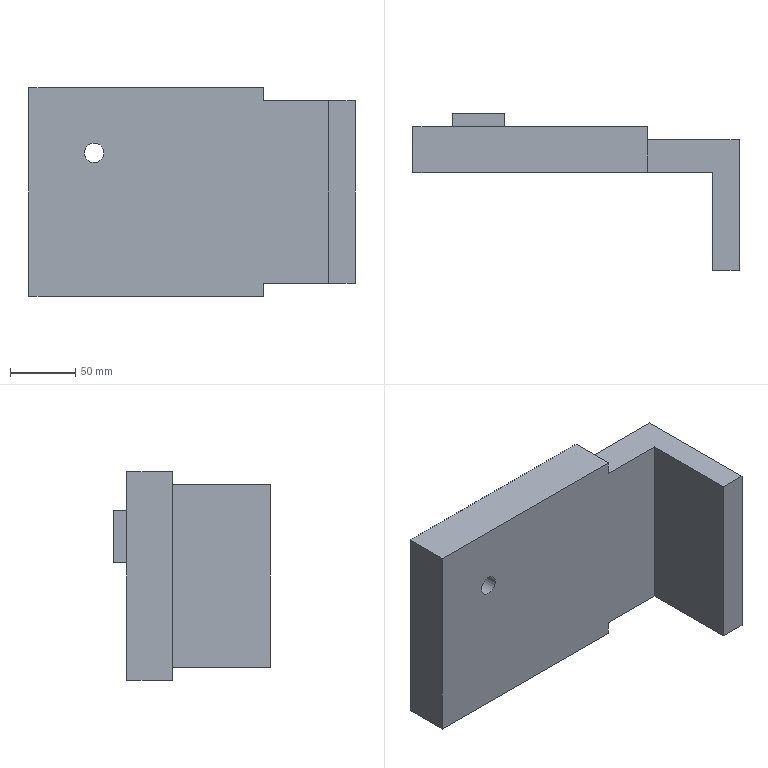Component | SolidWorks | MotorSupportPlate-1 | 1 solid | 19 faces | box 250 x 120 x 160 mm | volume 1471048 mm3 | plane 17 | cylinder 2 | commonest cylinder face diameters 15 x2
build123d program:
from build123d import *

# Parameters (mm, degrees)
SKETCH1_W                       = 20
SKETCH1_H                       = 140
BOSS_EXTRUDE1_DEPTH             = 100
SKETCH2_W                       = 25
SKETCH2_H                       = 140
BOSS_EXTRUDE2_DEPTH             = 230
BOSS_EXTRUDE3_REACH             = 482.755
SKETCH3_W                       = 180
SKETCH3_H                       = 160
BOSS_EXTRUDE3_DIRECTION_2_DEPTH = 10
SKETCH4_W                       = 40
SKETCH4_H                       = 40
SKETCH4_R                       = 7.5
BOSS_EXTRUDE4_DEPTH             = 10
CUT_EXTRUDE1_DEPTH              = 485.484
CUT_EXTRUDE1_DEPTH_BACK         = 485.484
SKETCH5_R                       = 7.5


with BuildPart() as part:
    # Sketch1 → Boss-Extrude1 (new body)
    with BuildSketch(Plane.XY):
        with Locations((455, 0)):
            Rectangle(SKETCH1_W, SKETCH1_H)
    extrude(amount=BOSS_EXTRUDE1_DEPTH)

    # Sketch2 → Boss-Extrude2 (add)
    with BuildSketch(Plane.ZY.offset(-445)):
        with Locations((87.5, 0)):
            Rectangle(SKETCH2_W, SKETCH2_H)
    extrude(amount=BOSS_EXTRUDE2_DEPTH)

    # Boss-Extrude3: up to this face of the body (flat: up to its plane)
    boss_extrude3_end = Plane(part.part.faces().sort_by_distance((330, 0, 75))[0])
    # Sketch3 → Boss-Extrude3 (add, up to the picked face)
    with BuildSketch(Plane.XY.offset(100), mode=Mode.PRIVATE) as boss_extrude3_sk1:
        with Locations((305, 0)):
            Rectangle(SKETCH3_W, SKETCH3_H)
    boss_extrude3_tool1 = split(extrude(boss_extrude3_sk1.sketch, amount=-BOSS_EXTRUDE3_REACH, mode=Mode.PRIVATE), bisect_by=boss_extrude3_end, keep=Keep.BOTH, mode=Mode.PRIVATE)
    add(boss_extrude3_tool1.solids().sort_by(Axis((305, 0, 100), (0, 0, -1)))[0])

    # Sketch3 → Boss-Extrude3 direction 2 (add)
    with BuildSketch(Plane.XY.offset(100)):
        with Locations((305, 0)):
            Rectangle(SKETCH3_W, SKETCH3_H)
    extrude(amount=BOSS_EXTRUDE3_DIRECTION_2_DEPTH)

    # Sketch4 → Boss-Extrude4 (add)
    with BuildSketch(Plane.XY.offset(110)):
        with Locations((265, -30)):
            Rectangle(SKETCH4_W, SKETCH4_H)
        with Locations((265, -30)):
            Circle(SKETCH4_R, mode=Mode.SUBTRACT)
    extrude(amount=BOSS_EXTRUDE4_DEPTH)

    # Sketch5 → Cut-Extrude1 (cut, two sides: drawn at the far end of the back side and taken through both)
    with BuildSketch(Plane.XY.offset(110).offset(-CUT_EXTRUDE1_DEPTH_BACK)):
        with Locations(Location((265, -30, 0), (0, 0, 270))):
            Circle(SKETCH5_R)
    extrude(amount=CUT_EXTRUDE1_DEPTH + CUT_EXTRUDE1_DEPTH_BACK, mode=Mode.SUBTRACT)


solid = part.part

# Placed as in the assembly
solid = solid.moved(Location((0, 150, 0), (-90, 0, 0)))
STEP:
#1=CARTESIAN_POINT('',(10.138,10.63,1.181));
#2=VERTEX_POINT('',#1);
#3=CARTESIAN_POINT('',(10.728,10.63,1.181));
#4=VERTEX_POINT('',#3);
#5=CARTESIAN_POINT('',(10.433,10.63,1.181));
#6=DIRECTION('',(0.,1.,0.));
#7=DIRECTION('',(1.,0.,0.));
#8=AXIS2_PLACEMENT_3D('',#5,#6,#7);
#9=CIRCLE('',#8,0.2953);
#10=EDGE_CURVE('',#2,#4,#9,.T.);
#11=ORIENTED_EDGE('',*,*,#10,.T.);
#12=CARTESIAN_POINT('',(10.728,8.858,1.181));
#13=VERTEX_POINT('',#12);
#14=CARTESIAN_POINT('',(10.728,10.63,1.181));
#15=DIRECTION('',(0.,-1.,0.));
#16=VECTOR('',#15,39.37);
#17=LINE('',#14,#16);
#18=EDGE_CURVE('',#4,#13,#17,.T.);
#19=ORIENTED_EDGE('',*,*,#18,.T.);
#20=CARTESIAN_POINT('',(10.138,8.858,1.181));
#21=VERTEX_POINT('',#20);
#22=CARTESIAN_POINT('',(10.433,8.858,1.181));
#23=DIRECTION('',(0.,1.,-0.));
#24=DIRECTION('',(0.,0.,1.));
#25=AXIS2_PLACEMENT_3D('',#22,#23,#24);
#26=CIRCLE('',#25,0.2953);
#27=EDGE_CURVE('',#21,#13,#26,.T.);
#28=ORIENTED_EDGE('',*,*,#27,.F.);
#29=CARTESIAN_POINT('',(10.138,10.63,1.181));
#30=DIRECTION('',(0.,-1.,0.));
#31=VECTOR('',#30,39.37);
#32=LINE('',#29,#31);
#33=EDGE_CURVE('',#2,#21,#32,.T.);
#34=ORIENTED_EDGE('',*,*,#33,.F.);
#35=EDGE_LOOP('',(#11,#19,#28,#34));
#36=FACE_OUTER_BOUND('',#35,.T.);
#37=CARTESIAN_POINT('',(10.433,10.63,1.181));
#38=DIRECTION('',(0.,-1.,0.));
#39=DIRECTION('',(-1.,0.,0.));
#40=AXIS2_PLACEMENT_3D('',#37,#38,#39);
#41=CYLINDRICAL_SURFACE('',#40,0.2953);
#42=ADVANCED_FACE('',(#36),#41,.F.);
#43=CARTESIAN_POINT('',(15.551,9.843,-2.756));
#44=VERTEX_POINT('',#43);
#45=CARTESIAN_POINT('',(15.551,8.858,-2.756));
#46=VERTEX_POINT('',#45);
#47=CARTESIAN_POINT('',(15.551,9.843,-2.756));
#48=DIRECTION('',(0.,-1.,0.));
#49=VECTOR('',#48,39.37);
#50=LINE('',#47,#49);
#51=EDGE_CURVE('',#44,#46,#50,.T.);
#52=ORIENTED_EDGE('',*,*,#51,.F.);
#53=CARTESIAN_POINT('',(18.307,9.843,-2.756));
#54=VERTEX_POINT('',#53);
#55=CARTESIAN_POINT('',(18.307,9.843,-2.756));
#56=DIRECTION('',(-1.,0.,0.));
#57=VECTOR('',#56,39.37);
#58=LINE('',#55,#57);
#59=EDGE_CURVE('',#54,#44,#58,.T.);
#60=ORIENTED_EDGE('',*,*,#59,.F.);
#61=CARTESIAN_POINT('',(18.307,5.906,-2.756));
#62=VERTEX_POINT('',#61);
#63=CARTESIAN_POINT('',(18.307,9.843,-2.756));
#64=DIRECTION('',(0.,-1.,0.));
#65=VECTOR('',#64,39.37);
#66=LINE('',#63,#65);
#67=EDGE_CURVE('',#54,#62,#66,.T.);
#68=ORIENTED_EDGE('',*,*,#67,.T.);
#69=CARTESIAN_POINT('',(17.52,5.906,-2.756));
#70=VERTEX_POINT('',#69);
#71=CARTESIAN_POINT('',(18.307,5.906,-2.756));
#72=DIRECTION('',(-1.,0.,0.));
#73=VECTOR('',#72,39.37);
#74=LINE('',#71,#73);
#75=EDGE_CURVE('',#62,#70,#74,.T.);
#76=ORIENTED_EDGE('',*,*,#75,.T.);
#77=CARTESIAN_POINT('',(17.52,8.858,-2.756));
#78=VERTEX_POINT('',#77);
#79=CARTESIAN_POINT('',(17.52,9.843,-2.756));
#80=DIRECTION('',(0.,-1.,0.));
#81=VECTOR('',#80,39.37);
#82=LINE('',#79,#81);
#83=EDGE_CURVE('',#78,#70,#82,.T.);
#84=ORIENTED_EDGE('',*,*,#83,.F.);
#85=CARTESIAN_POINT('',(8.465,8.858,-2.756));
#86=DIRECTION('',(1.,0.,0.));
#87=VECTOR('',#86,39.37);
#88=LINE('',#85,#87);
#89=EDGE_CURVE('',#46,#78,#88,.T.);
#90=ORIENTED_EDGE('',*,*,#89,.F.);
#91=EDGE_LOOP('',(#52,#60,#68,#76,#84,#90));
#92=FACE_OUTER_BOUND('',#91,.T.);
#93=CARTESIAN_POINT('',(18.307,9.843,-2.756));
#94=DIRECTION('',(0.,0.,1.));
#95=DIRECTION('',(0.,-1.,0.));
#96=AXIS2_PLACEMENT_3D('',#93,#94,#95);
#97=PLANE('',#96);
#98=ADVANCED_FACE('',(#92),#97,.F.);
#99=CARTESIAN_POINT('',(15.551,8.858,2.756));
#100=VERTEX_POINT('',#99);
#101=CARTESIAN_POINT('',(15.551,9.843,2.756));
#102=VERTEX_POINT('',#101);
#103=CARTESIAN_POINT('',(15.551,9.843,2.756));
#104=DIRECTION('',(0.,1.,0.));
#105=VECTOR('',#104,39.37);
#106=LINE('',#103,#105);
#107=EDGE_CURVE('',#100,#102,#106,.T.);
#108=ORIENTED_EDGE('',*,*,#107,.F.);
#109=CARTESIAN_POINT('',(17.52,8.858,2.756));
#110=VERTEX_POINT('',#109);
#111=CARTESIAN_POINT('',(8.465,8.858,2.756));
#112=DIRECTION('',(1.,0.,0.));
#113=VECTOR('',#112,39.37);
#114=LINE('',#111,#113);
#115=EDGE_CURVE('',#100,#110,#114,.T.);
#116=ORIENTED_EDGE('',*,*,#115,.T.);
#117=CARTESIAN_POINT('',(17.52,5.906,2.756));
#118=VERTEX_POINT('',#117);
#119=CARTESIAN_POINT('',(17.52,9.843,2.756));
#120=DIRECTION('',(0.,-1.,0.));
#121=VECTOR('',#120,39.37);
#122=LINE('',#119,#121);
#123=EDGE_CURVE('',#110,#118,#122,.T.);
#124=ORIENTED_EDGE('',*,*,#123,.T.);
#125=CARTESIAN_POINT('',(18.307,5.906,2.756));
#126=VERTEX_POINT('',#125);
#127=CARTESIAN_POINT('',(18.307,5.906,2.756));
#128=DIRECTION('',(1.,0.,0.));
#129=VECTOR('',#128,39.37);
#130=LINE('',#127,#129);
#131=EDGE_CURVE('',#118,#126,#130,.T.);
#132=ORIENTED_EDGE('',*,*,#131,.T.);
#133=CARTESIAN_POINT('',(18.307,9.843,2.756));
#134=VERTEX_POINT('',#133);
#135=CARTESIAN_POINT('',(18.307,9.843,2.756));
#136=DIRECTION('',(0.,-1.,0.));
#137=VECTOR('',#136,39.37);
#138=LINE('',#135,#137);
#139=EDGE_CURVE('',#134,#126,#138,.T.);
#140=ORIENTED_EDGE('',*,*,#139,.F.);
#141=CARTESIAN_POINT('',(18.307,9.843,2.756));
#142=DIRECTION('',(1.,0.,0.));
#143=VECTOR('',#142,39.37);
#144=LINE('',#141,#143);
#145=EDGE_CURVE('',#102,#134,#144,.T.);
#146=ORIENTED_EDGE('',*,*,#145,.F.);
#147=EDGE_LOOP('',(#108,#116,#124,#132,#140,#146));
#148=FACE_OUTER_BOUND('',#147,.T.);
#149=CARTESIAN_POINT('',(18.307,9.843,2.756));
#150=DIRECTION('',(0.,0.,-1.));
#151=DIRECTION('',(-1.,0.,-0.));
#152=AXIS2_PLACEMENT_3D('',#149,#150,#151);
#153=PLANE('',#152);
#154=ADVANCED_FACE('',(#148),#153,.F.);
#155=ORIENTED_EDGE('',*,*,#59,.T.);
#156=CARTESIAN_POINT('',(15.551,9.843,0.));
#157=DIRECTION('',(0.,0.,1.));
#158=VECTOR('',#157,39.37);
#159=LINE('',#156,#158);
#160=EDGE_CURVE('',#44,#102,#159,.T.);
#161=ORIENTED_EDGE('',*,*,#160,.T.);
#162=ORIENTED_EDGE('',*,*,#145,.T.);
#163=CARTESIAN_POINT('',(18.307,9.843,2.756));
#164=DIRECTION('',(0.,0.,-1.));
#165=VECTOR('',#164,39.37);
#166=LINE('',#163,#165);
#167=EDGE_CURVE('',#134,#54,#166,.T.);
#168=ORIENTED_EDGE('',*,*,#167,.T.);
#169=EDGE_LOOP('',(#155,#161,#162,#168));
#170=FACE_OUTER_BOUND('',#169,.T.);
#171=CARTESIAN_POINT('',(0.,9.843,0.));
#172=DIRECTION('',(0.,1.,0.));
#173=DIRECTION('',(1.,0.,0.));
#174=AXIS2_PLACEMENT_3D('',#171,#172,#173);
#175=PLANE('',#174);
#176=ADVANCED_FACE('',(#170),#175,.T.);
#177=CARTESIAN_POINT('',(17.52,8.858,-2.756));
#178=DIRECTION('',(0.,0.,1.));
#179=VECTOR('',#178,39.37);
#180=LINE('',#177,#179);
#181=EDGE_CURVE('',#78,#110,#180,.T.);
#182=ORIENTED_EDGE('',*,*,#181,.F.);
#183=ORIENTED_EDGE('',*,*,#83,.T.);
#184=CARTESIAN_POINT('',(17.52,5.906,2.756));
#185=DIRECTION('',(0.,0.,1.));
#186=VECTOR('',#185,39.37);
#187=LINE('',#184,#186);
#188=EDGE_CURVE('',#70,#118,#187,.T.);
#189=ORIENTED_EDGE('',*,*,#188,.T.);
#190=ORIENTED_EDGE('',*,*,#123,.F.);
#191=EDGE_LOOP('',(#182,#183,#189,#190));
#192=FACE_OUTER_BOUND('',#191,.T.);
#193=CARTESIAN_POINT('',(17.52,9.843,2.756));
#194=DIRECTION('',(1.,0.,0.));
#195=DIRECTION('',(0.,-1.,0.));
#196=AXIS2_PLACEMENT_3D('',#193,#194,#195);
#197=PLANE('',#196);
#198=ADVANCED_FACE('',(#192),#197,.F.);
#199=CARTESIAN_POINT('',(18.307,5.906,2.756));
#200=DIRECTION('',(0.,0.,-1.));
#201=VECTOR('',#200,39.37);
#202=LINE('',#199,#201);
#203=EDGE_CURVE('',#126,#62,#202,.T.);
#204=ORIENTED_EDGE('',*,*,#203,.T.);
#205=ORIENTED_EDGE('',*,*,#67,.F.);
#206=ORIENTED_EDGE('',*,*,#167,.F.);
#207=ORIENTED_EDGE('',*,*,#139,.T.);
#208=EDGE_LOOP('',(#204,#205,#206,#207));
#209=FACE_OUTER_BOUND('',#208,.T.);
#210=CARTESIAN_POINT('',(18.307,9.843,2.756));
#211=DIRECTION('',(-1.,0.,0.));
#212=DIRECTION('',(0.,1.,0.));
#213=AXIS2_PLACEMENT_3D('',#210,#211,#212);
#214=PLANE('',#213);
#215=ADVANCED_FACE('',(#209),#214,.F.);
#216=ORIENTED_EDGE('',*,*,#203,.F.);
#217=ORIENTED_EDGE('',*,*,#131,.F.);
#218=ORIENTED_EDGE('',*,*,#188,.F.);
#219=ORIENTED_EDGE('',*,*,#75,.F.);
#220=EDGE_LOOP('',(#216,#217,#218,#219));
#221=FACE_OUTER_BOUND('',#220,.T.);
#222=CARTESIAN_POINT('',(0.,5.906,0.));
#223=DIRECTION('',(0.,1.,0.));
#224=DIRECTION('',(1.,0.,0.));
#225=AXIS2_PLACEMENT_3D('',#222,#223,#224);
#226=PLANE('',#225);
#227=ADVANCED_FACE('',(#221),#226,.F.);
#228=ORIENTED_EDGE('',*,*,#27,.T.);
#229=CARTESIAN_POINT('',(10.433,8.858,1.181));
#230=DIRECTION('',(0.,1.,-0.));
#231=DIRECTION('',(0.,0.,1.));
#232=AXIS2_PLACEMENT_3D('',#229,#230,#231);
#233=CIRCLE('',#232,0.2953);
#234=EDGE_CURVE('',#13,#21,#233,.T.);
#235=ORIENTED_EDGE('',*,*,#234,.T.);
#236=EDGE_LOOP('',(#228,#235));
#237=FACE_BOUND('',#236,.T.);
#238=CARTESIAN_POINT('',(8.465,8.858,-3.15));
#239=VERTEX_POINT('',#238);
#240=CARTESIAN_POINT('',(8.465,8.858,3.15));
#241=VERTEX_POINT('',#240);
#242=CARTESIAN_POINT('',(8.465,8.858,-2.756));
#243=DIRECTION('',(0.,0.,1.));
#244=VECTOR('',#243,39.37);
#245=LINE('',#242,#244);
#246=EDGE_CURVE('',#239,#241,#245,.T.);
#247=ORIENTED_EDGE('',*,*,#246,.F.);
#248=CARTESIAN_POINT('',(15.551,8.858,-3.15));
#249=VERTEX_POINT('',#248);
#250=CARTESIAN_POINT('',(8.465,8.858,-3.15));
#251=DIRECTION('',(1.,0.,0.));
#252=VECTOR('',#251,39.37);
#253=LINE('',#250,#252);
#254=EDGE_CURVE('',#239,#249,#253,.T.);
#255=ORIENTED_EDGE('',*,*,#254,.T.);
#256=CARTESIAN_POINT('',(15.551,8.858,-3.15));
#257=DIRECTION('',(0.,0.,1.));
#258=VECTOR('',#257,39.37);
#259=LINE('',#256,#258);
#260=EDGE_CURVE('',#249,#46,#259,.T.);
#261=ORIENTED_EDGE('',*,*,#260,.T.);
#262=ORIENTED_EDGE('',*,*,#89,.T.);
#263=ORIENTED_EDGE('',*,*,#181,.T.);
#264=ORIENTED_EDGE('',*,*,#115,.F.);
#265=CARTESIAN_POINT('',(15.551,8.858,3.15));
#266=VERTEX_POINT('',#265);
#267=CARTESIAN_POINT('',(15.551,8.858,-3.15));
#268=DIRECTION('',(0.,0.,1.));
#269=VECTOR('',#268,39.37);
#270=LINE('',#267,#269);
#271=EDGE_CURVE('',#100,#266,#270,.T.);
#272=ORIENTED_EDGE('',*,*,#271,.T.);
#273=CARTESIAN_POINT('',(8.465,8.858,3.15));
#274=DIRECTION('',(-1.,0.,0.));
#275=VECTOR('',#274,39.37);
#276=LINE('',#273,#275);
#277=EDGE_CURVE('',#266,#241,#276,.T.);
#278=ORIENTED_EDGE('',*,*,#277,.T.);
#279=EDGE_LOOP('',(#247,#255,#261,#262,#263,#264,#272,#278));
#280=FACE_OUTER_BOUND('',#279,.T.);
#281=CARTESIAN_POINT('',(8.465,8.858,-2.756));
#282=DIRECTION('',(0.,1.,-0.));
#283=DIRECTION('',(0.,0.,1.));
#284=AXIS2_PLACEMENT_3D('',#281,#282,#283);
#285=PLANE('',#284);
#286=ADVANCED_FACE('',(#237,#280),#285,.F.);
#287=CARTESIAN_POINT('',(8.465,10.236,-3.15));
#288=VERTEX_POINT('',#287);
#289=CARTESIAN_POINT('',(8.465,10.236,-3.15));
#290=DIRECTION('',(0.,-1.,0.));
#291=VECTOR('',#290,39.37);
#292=LINE('',#289,#291);
#293=EDGE_CURVE('',#288,#239,#292,.T.);
#294=ORIENTED_EDGE('',*,*,#293,.T.);
#295=ORIENTED_EDGE('',*,*,#246,.T.);
#296=CARTESIAN_POINT('',(8.465,10.236,3.15));
#297=VERTEX_POINT('',#296);
#298=CARTESIAN_POINT('',(8.465,10.236,3.15));
#299=DIRECTION('',(0.,-1.,0.));
#300=VECTOR('',#299,39.37);
#301=LINE('',#298,#300);
#302=EDGE_CURVE('',#297,#241,#301,.T.);
#303=ORIENTED_EDGE('',*,*,#302,.F.);
#304=CARTESIAN_POINT('',(8.465,10.236,-3.15));
#305=DIRECTION('',(0.,0.,1.));
#306=VECTOR('',#305,39.37);
#307=LINE('',#304,#306);
#308=EDGE_CURVE('',#288,#297,#307,.T.);
#309=ORIENTED_EDGE('',*,*,#308,.F.);
#310=EDGE_LOOP('',(#294,#295,#303,#309));
#311=FACE_OUTER_BOUND('',#310,.T.);
#312=CARTESIAN_POINT('',(8.465,5.906,0.));
#313=DIRECTION('',(1.,0.,0.));
#314=DIRECTION('',(0.,-1.,0.));
#315=AXIS2_PLACEMENT_3D('',#312,#313,#314);
#316=PLANE('',#315);
#317=ADVANCED_FACE('',(#311),#316,.F.);
#318=ORIENTED_EDGE('',*,*,#160,.F.);
#319=ORIENTED_EDGE('',*,*,#51,.T.);
#320=ORIENTED_EDGE('',*,*,#260,.F.);
#321=CARTESIAN_POINT('',(15.551,10.236,-3.15));
#322=VERTEX_POINT('',#321);
#323=CARTESIAN_POINT('',(15.551,10.236,-3.15));
#324=DIRECTION('',(0.,-1.,0.));
#325=VECTOR('',#324,39.37);
#326=LINE('',#323,#325);
#327=EDGE_CURVE('',#322,#249,#326,.T.);
#328=ORIENTED_EDGE('',*,*,#327,.F.);
#329=CARTESIAN_POINT('',(15.551,10.236,3.15));
#330=VERTEX_POINT('',#329);
#331=CARTESIAN_POINT('',(15.551,10.236,-3.15));
#332=DIRECTION('',(0.,0.,-1.));
#333=VECTOR('',#332,39.37);
#334=LINE('',#331,#333);
#335=EDGE_CURVE('',#330,#322,#334,.T.);
#336=ORIENTED_EDGE('',*,*,#335,.F.);
#337=CARTESIAN_POINT('',(15.551,10.236,3.15));
#338=DIRECTION('',(0.,-1.,0.));
#339=VECTOR('',#338,39.37);
#340=LINE('',#337,#339);
#341=EDGE_CURVE('',#330,#266,#340,.T.);
#342=ORIENTED_EDGE('',*,*,#341,.T.);
#343=ORIENTED_EDGE('',*,*,#271,.F.);
#344=ORIENTED_EDGE('',*,*,#107,.T.);
#345=EDGE_LOOP('',(#318,#319,#320,#328,#336,#342,#343,#344));
#346=FACE_OUTER_BOUND('',#345,.T.);
#347=CARTESIAN_POINT('',(15.551,10.236,-3.15));
#348=DIRECTION('',(-1.,0.,0.));
#349=DIRECTION('',(0.,1.,0.));
#350=AXIS2_PLACEMENT_3D('',#347,#348,#349);
#351=PLANE('',#350);
#352=ADVANCED_FACE('',(#346),#351,.F.);
#353=ORIENTED_EDGE('',*,*,#302,.T.);
#354=ORIENTED_EDGE('',*,*,#277,.F.);
#355=ORIENTED_EDGE('',*,*,#341,.F.);
#356=CARTESIAN_POINT('',(8.465,10.236,3.15));
#357=DIRECTION('',(1.,0.,-0.));
#358=VECTOR('',#357,39.37);
#359=LINE('',#356,#358);
#360=EDGE_CURVE('',#297,#330,#359,.T.);
#361=ORIENTED_EDGE('',*,*,#360,.F.);
#362=EDGE_LOOP('',(#353,#354,#355,#361));
#363=FACE_OUTER_BOUND('',#362,.T.);
#364=CARTESIAN_POINT('',(8.465,10.236,3.15));
#365=DIRECTION('',(-0.,0.,-1.));
#366=DIRECTION('',(-1.,0.,0.));
#367=AXIS2_PLACEMENT_3D('',#364,#365,#366);
#368=PLANE('',#367);
#369=ADVANCED_FACE('',(#363),#368,.F.);
#370=ORIENTED_EDGE('',*,*,#327,.T.);
#371=ORIENTED_EDGE('',*,*,#254,.F.);
#372=ORIENTED_EDGE('',*,*,#293,.F.);
#373=CARTESIAN_POINT('',(8.465,10.236,-3.15));
#374=DIRECTION('',(-1.,0.,0.));
#375=VECTOR('',#374,39.37);
#376=LINE('',#373,#375);
#377=EDGE_CURVE('',#322,#288,#376,.T.);
#378=ORIENTED_EDGE('',*,*,#377,.F.);
#379=EDGE_LOOP('',(#370,#371,#372,#378));
#380=FACE_OUTER_BOUND('',#379,.T.);
#381=CARTESIAN_POINT('',(8.465,10.236,-3.15));
#382=DIRECTION('',(0.,0.,1.));
#383=DIRECTION('',(0.,-1.,0.));
#384=AXIS2_PLACEMENT_3D('',#381,#382,#383);
#385=PLANE('',#384);
#386=ADVANCED_FACE('',(#380),#385,.F.);
#387=CARTESIAN_POINT('',(11.22,10.236,0.3937));
#388=VERTEX_POINT('',#387);
#389=CARTESIAN_POINT('',(9.646,10.236,0.3937));
#390=VERTEX_POINT('',#389);
#391=CARTESIAN_POINT('',(9.646,10.236,0.3937));
#392=DIRECTION('',(-1.,0.,0.));
#393=VECTOR('',#392,39.37);
#394=LINE('',#391,#393);
#395=EDGE_CURVE('',#388,#390,#394,.T.);
#396=ORIENTED_EDGE('',*,*,#395,.F.);
#397=CARTESIAN_POINT('',(11.22,10.236,1.969));
#398=VERTEX_POINT('',#397);
#399=CARTESIAN_POINT('',(11.22,10.236,0.3937));
#400=DIRECTION('',(0.,0.,-1.));
#401=VECTOR('',#400,39.37);
#402=LINE('',#399,#401);
#403=EDGE_CURVE('',#398,#388,#402,.T.);
#404=ORIENTED_EDGE('',*,*,#403,.F.);
#405=CARTESIAN_POINT('',(9.646,10.236,1.969));
#406=VERTEX_POINT('',#405);
#407=CARTESIAN_POINT('',(9.646,10.236,1.969));
#408=DIRECTION('',(1.,0.,0.));
#409=VECTOR('',#408,39.37);
#410=LINE('',#407,#409);
#411=EDGE_CURVE('',#406,#398,#410,.T.);
#412=ORIENTED_EDGE('',*,*,#411,.F.);
#413=CARTESIAN_POINT('',(9.646,10.236,0.3937));
#414=DIRECTION('',(0.,0.,1.));
#415=VECTOR('',#414,39.37);
#416=LINE('',#413,#415);
#417=EDGE_CURVE('',#390,#406,#416,.T.);
#418=ORIENTED_EDGE('',*,*,#417,.F.);
#419=EDGE_LOOP('',(#396,#404,#412,#418));
#420=FACE_BOUND('',#419,.T.);
#421=ORIENTED_EDGE('',*,*,#308,.T.);
#422=ORIENTED_EDGE('',*,*,#360,.T.);
#423=ORIENTED_EDGE('',*,*,#335,.T.);
#424=ORIENTED_EDGE('',*,*,#377,.T.);
#425=EDGE_LOOP('',(#421,#422,#423,#424));
#426=FACE_OUTER_BOUND('',#425,.T.);
#427=CARTESIAN_POINT('',(0.,10.236,0.));
#428=DIRECTION('',(0.,1.,0.));
#429=DIRECTION('',(1.,0.,0.));
#430=AXIS2_PLACEMENT_3D('',#427,#428,#429);
#431=PLANE('',#430);
#432=ADVANCED_FACE('',(#420,#426),#431,.T.);
#433=CARTESIAN_POINT('',(11.22,10.63,1.969));
#434=VERTEX_POINT('',#433);
#435=CARTESIAN_POINT('',(11.22,10.63,0.3937));
#436=VERTEX_POINT('',#435);
#437=CARTESIAN_POINT('',(11.22,10.63,0.3937));
#438=DIRECTION('',(0.,0.,-1.));
#439=VECTOR('',#438,39.37);
#440=LINE('',#437,#439);
#441=EDGE_CURVE('',#434,#436,#440,.T.);
#442=ORIENTED_EDGE('',*,*,#441,.T.);
#443=CARTESIAN_POINT('',(9.646,10.63,0.3937));
#444=VERTEX_POINT('',#443);
#445=CARTESIAN_POINT('',(9.646,10.63,0.3937));
#446=DIRECTION('',(-1.,0.,0.));
#447=VECTOR('',#446,39.37);
#448=LINE('',#445,#447);
#449=EDGE_CURVE('',#436,#444,#448,.T.);
#450=ORIENTED_EDGE('',*,*,#449,.T.);
#451=CARTESIAN_POINT('',(9.646,10.63,1.969));
#452=VERTEX_POINT('',#451);
#453=CARTESIAN_POINT('',(9.646,10.63,0.3937));
#454=DIRECTION('',(0.,0.,1.));
#455=VECTOR('',#454,39.37);
#456=LINE('',#453,#455);
#457=EDGE_CURVE('',#444,#452,#456,.T.);
#458=ORIENTED_EDGE('',*,*,#457,.T.);
#459=CARTESIAN_POINT('',(9.646,10.63,1.969));
#460=DIRECTION('',(1.,0.,0.));
#461=VECTOR('',#460,39.37);
#462=LINE('',#459,#461);
#463=EDGE_CURVE('',#452,#434,#462,.T.);
#464=ORIENTED_EDGE('',*,*,#463,.T.);
#465=EDGE_LOOP('',(#442,#450,#458,#464));
#466=FACE_OUTER_BOUND('',#465,.T.);
#467=ORIENTED_EDGE('',*,*,#10,.F.);
#468=CARTESIAN_POINT('',(10.433,10.63,1.181));
#469=DIRECTION('',(0.,1.,0.));
#470=DIRECTION('',(1.,0.,0.));
#471=AXIS2_PLACEMENT_3D('',#468,#469,#470);
#472=CIRCLE('',#471,0.2953);
#473=EDGE_CURVE('',#4,#2,#472,.T.);
#474=ORIENTED_EDGE('',*,*,#473,.F.);
#475=EDGE_LOOP('',(#467,#474));
#476=FACE_BOUND('',#475,.T.);
#477=CARTESIAN_POINT('',(0.,10.63,0.));
#478=DIRECTION('',(0.,1.,0.));
#479=DIRECTION('',(1.,0.,0.));
#480=AXIS2_PLACEMENT_3D('',#477,#478,#479);
#481=PLANE('',#480);
#482=ADVANCED_FACE('',(#466,#476),#481,.T.);
#483=ORIENTED_EDGE('',*,*,#403,.T.);
#484=CARTESIAN_POINT('',(11.22,10.63,0.3937));
#485=DIRECTION('',(0.,-1.,0.));
#486=VECTOR('',#485,39.37);
#487=LINE('',#484,#486);
#488=EDGE_CURVE('',#436,#388,#487,.T.);
#489=ORIENTED_EDGE('',*,*,#488,.F.);
#490=ORIENTED_EDGE('',*,*,#441,.F.);
#491=CARTESIAN_POINT('',(11.22,10.63,1.969));
#492=DIRECTION('',(0.,-1.,0.));
#493=VECTOR('',#492,39.37);
#494=LINE('',#491,#493);
#495=EDGE_CURVE('',#434,#398,#494,.T.);
#496=ORIENTED_EDGE('',*,*,#495,.T.);
#497=EDGE_LOOP('',(#483,#489,#490,#496));
#498=FACE_OUTER_BOUND('',#497,.T.);
#499=CARTESIAN_POINT('',(11.22,10.63,0.3937));
#500=DIRECTION('',(-1.,0.,0.));
#501=DIRECTION('',(0.,1.,0.));
#502=AXIS2_PLACEMENT_3D('',#499,#500,#501);
#503=PLANE('',#502);
#504=ADVANCED_FACE('',(#498),#503,.F.);
#505=ORIENTED_EDGE('',*,*,#395,.T.);
#506=CARTESIAN_POINT('',(9.646,10.63,0.3937));
#507=DIRECTION('',(0.,-1.,0.));
#508=VECTOR('',#507,39.37);
#509=LINE('',#506,#508);
#510=EDGE_CURVE('',#444,#390,#509,.T.);
#511=ORIENTED_EDGE('',*,*,#510,.F.);
#512=ORIENTED_EDGE('',*,*,#449,.F.);
#513=ORIENTED_EDGE('',*,*,#488,.T.);
#514=EDGE_LOOP('',(#505,#511,#512,#513));
#515=FACE_OUTER_BOUND('',#514,.T.);
#516=CARTESIAN_POINT('',(9.646,10.63,0.3937));
#517=DIRECTION('',(0.,0.,1.));
#518=DIRECTION('',(1.,0.,-0.));
#519=AXIS2_PLACEMENT_3D('',#516,#517,#518);
#520=PLANE('',#519);
#521=ADVANCED_FACE('',(#515),#520,.F.);
#522=ORIENTED_EDGE('',*,*,#417,.T.);
#523=CARTESIAN_POINT('',(9.646,10.63,1.969));
#524=DIRECTION('',(0.,-1.,0.));
#525=VECTOR('',#524,39.37);
#526=LINE('',#523,#525);
#527=EDGE_CURVE('',#452,#406,#526,.T.);
#528=ORIENTED_EDGE('',*,*,#527,.F.);
#529=ORIENTED_EDGE('',*,*,#457,.F.);
#530=ORIENTED_EDGE('',*,*,#510,.T.);
#531=EDGE_LOOP('',(#522,#528,#529,#530));
#532=FACE_OUTER_BOUND('',#531,.T.);
#533=CARTESIAN_POINT('',(9.646,10.63,0.3937));
#534=DIRECTION('',(1.,0.,0.));
#535=DIRECTION('',(0.,-1.,0.));
#536=AXIS2_PLACEMENT_3D('',#533,#534,#535);
#537=PLANE('',#536);
#538=ADVANCED_FACE('',(#532),#537,.F.);
#539=ORIENTED_EDGE('',*,*,#411,.T.);
#540=ORIENTED_EDGE('',*,*,#495,.F.);
#541=ORIENTED_EDGE('',*,*,#463,.F.);
#542=ORIENTED_EDGE('',*,*,#527,.T.);
#543=EDGE_LOOP('',(#539,#540,#541,#542));
#544=FACE_OUTER_BOUND('',#543,.T.);
#545=CARTESIAN_POINT('',(9.646,10.63,1.969));
#546=DIRECTION('',(0.,0.,-1.));
#547=DIRECTION('',(0.,1.,0.));
#548=AXIS2_PLACEMENT_3D('',#545,#546,#547);
#549=PLANE('',#548);
#550=ADVANCED_FACE('',(#544),#549,.F.);
#551=ORIENTED_EDGE('',*,*,#18,.F.);
#552=ORIENTED_EDGE('',*,*,#473,.T.);
#553=ORIENTED_EDGE('',*,*,#33,.T.);
#554=ORIENTED_EDGE('',*,*,#234,.F.);
#555=EDGE_LOOP('',(#551,#552,#553,#554));
#556=FACE_OUTER_BOUND('',#555,.T.);
#557=CARTESIAN_POINT('',(10.433,10.63,1.181));
#558=DIRECTION('',(0.,-1.,0.));
#559=DIRECTION('',(-1.,0.,0.));
#560=AXIS2_PLACEMENT_3D('',#557,#558,#559);
#561=CYLINDRICAL_SURFACE('',#560,0.2953);
#562=ADVANCED_FACE('',(#556),#561,.F.);
#563=CLOSED_SHELL('',(#42,#98,#154,#176,#198,#215,#227,#286,#317,#352,#369,#386,#432,#482,#504,#521,#538,#550,#562));
#564=MANIFOLD_SOLID_BREP('',#563);
#565=CARTESIAN_POINT('',(0.,0.,0.));
#566=DIRECTION('',(0.,0.,1.));
#567=DIRECTION('',(1.,0.,0.));
#568=AXIS2_PLACEMENT_3D('',#565,#566,#567);
#569=(LENGTH_UNIT()NAMED_UNIT(*)SI_UNIT($,.METRE.));
#570=LENGTH_MEASURE_WITH_UNIT(LENGTH_MEASURE(0.0254),#569);
#571=DIMENSIONAL_EXPONENTS(1.,0.,0.,0.,0.,0.,0.);
#572=(CONVERSION_BASED_UNIT('',#570)LENGTH_UNIT()NAMED_UNIT(#571));
#573=UNCERTAINTY_MEASURE_WITH_UNIT(LENGTH_MEASURE(0.00001),#572,'','');
#574=(NAMED_UNIT(*)PLANE_ANGLE_UNIT()SI_UNIT($,.RADIAN.));
#575=(NAMED_UNIT(*)SI_UNIT($,.STERADIAN.)SOLID_ANGLE_UNIT());
#576=(GEOMETRIC_REPRESENTATION_CONTEXT(3)GLOBAL_UNCERTAINTY_ASSIGNED_CONTEXT((#573))GLOBAL_UNIT_ASSIGNED_CONTEXT((#572,#574,#575))REPRESENTATION_CONTEXT('',''));
#577=ADVANCED_BREP_SHAPE_REPRESENTATION('',(#564,#568),#576);
#578=COLOUR_RGB('',0.7922,0.8196,0.9333);
#579=FILL_AREA_STYLE_COLOUR('',#578);
#580=FILL_AREA_STYLE('',(#579));
#581=SURFACE_STYLE_FILL_AREA(#580);
#582=SURFACE_SIDE_STYLE('',(#581));
#583=SURFACE_STYLE_USAGE(.BOTH.,#582);
#584=PRESENTATION_STYLE_ASSIGNMENT((#583));
#585=STYLED_ITEM('',(#584),#564);
#586=PRESENTATION_LAYER_ASSIGNMENT('','',(#585));
#587=(LENGTH_UNIT()NAMED_UNIT(*)SI_UNIT($,.METRE.));
#588=LENGTH_MEASURE_WITH_UNIT(LENGTH_MEASURE(0.0254),#587);
#589=DIMENSIONAL_EXPONENTS(1.,0.,0.,0.,0.,0.,0.);
#590=(CONVERSION_BASED_UNIT('',#588)LENGTH_UNIT()NAMED_UNIT(#589));
#591=UNCERTAINTY_MEASURE_WITH_UNIT(LENGTH_MEASURE(0.00001),#590,'','');
#592=(NAMED_UNIT(*)PLANE_ANGLE_UNIT()SI_UNIT($,.RADIAN.));
#593=(NAMED_UNIT(*)SI_UNIT($,.STERADIAN.)SOLID_ANGLE_UNIT());
#594=(GEOMETRIC_REPRESENTATION_CONTEXT(3)GLOBAL_UNCERTAINTY_ASSIGNED_CONTEXT((#591))GLOBAL_UNIT_ASSIGNED_CONTEXT((#590,#592,#593))REPRESENTATION_CONTEXT('',''));
#595=MECHANICAL_DESIGN_GEOMETRIC_PRESENTATION_REPRESENTATION('',(#585),#594);